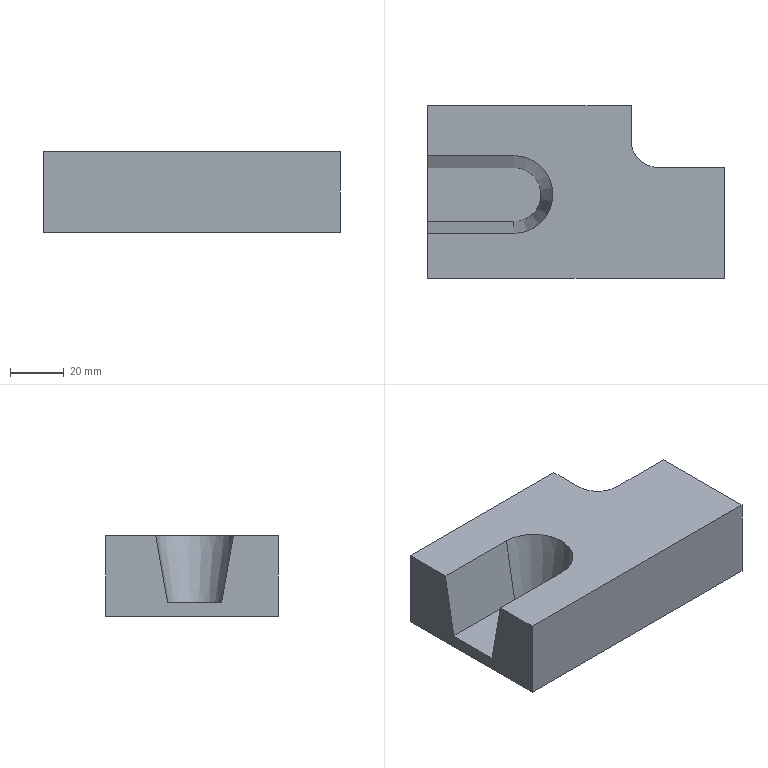CAM job | NX | mm | 3-axis | 1 set-up | 1 operations | part box 110 x 64 x 30
set-up 1
1. Cavity Milling | Mill Mill5 D16 | CAVITY_MILL | path 11681.387 mm | 31.134 min